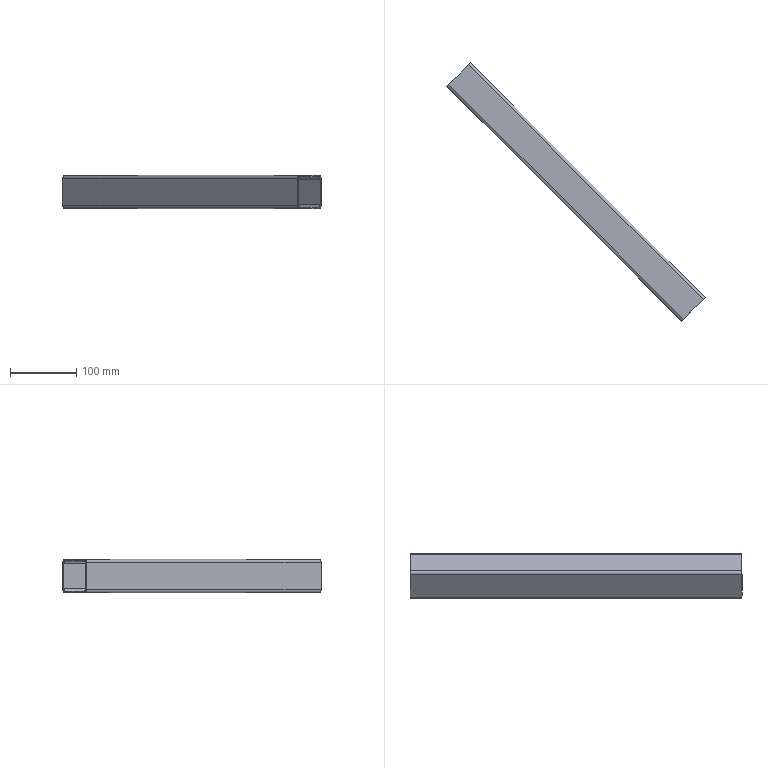Component | NX | SLID_FRAME_BOT_BEAM | 1 solid | 18 faces | volume 192000 mm3 | plane 10 | cylinder 8 | commonest cylinder face diameters 8 x8